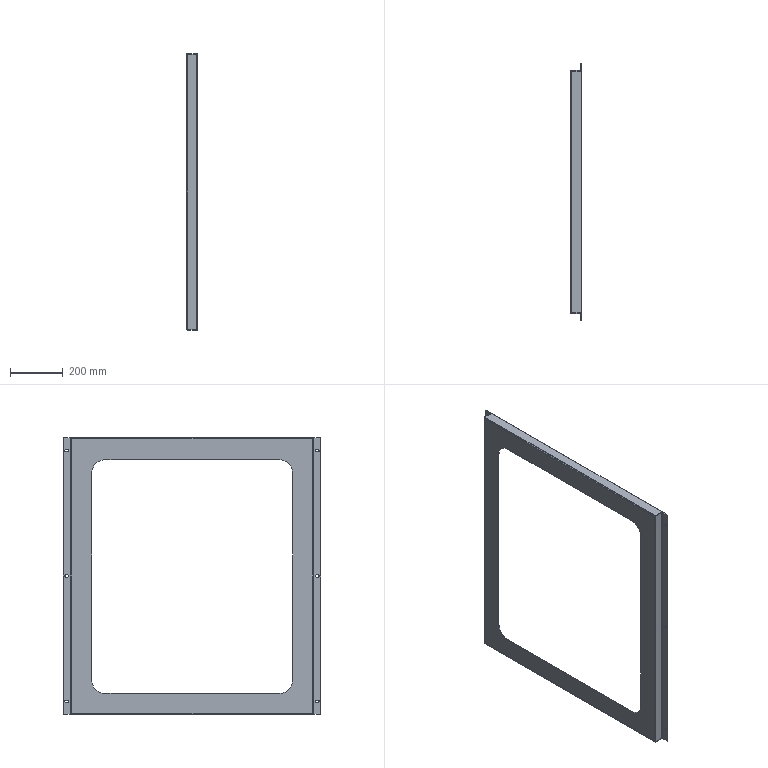Component | SolidWorks | ExhaustVentAssembly-1_ExhaustVent-1 | 1 solid | 92 faces | volume 985426 mm3 | plane 50 | cylinder 34 | spline 8 | commonest cylinder face diameters 9.5 x18 4 x6 8 x6 100 x4 | material Plain Carbon Steel